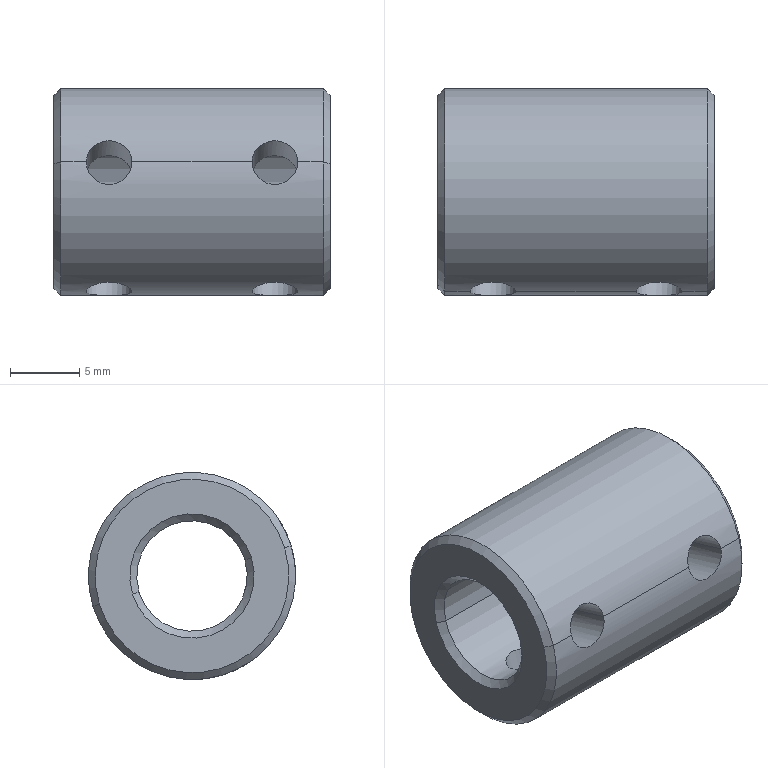Component | SolidWorks | 04-004CouplingSleeve-1 | 1 solid | 22 faces | box 20 x 15 x 15 mm | volume 2390 mm3 | cylinder 12 | cone 8 | plane 2 | commonest cylinder face diameters 3.3 x8 8 x2 15 x2
build123d program:
from build123d import *

# Parameters (mm, degrees)
SKETCH1_R             = 7.5
SKETCH1_R_2           = 4
BOSS_EXTRUDE1_DEPTH   = 20
M4_TAPPED_HOLE1_D     = 3.3
M4_TAPPED_HOLE1_DEPTH = 6
M4_TAPPED_HOLE1_TIP   = 0.9914
M4_TAPPED_HOLE2_D     = 3.3
M4_TAPPED_HOLE2_DEPTH = 10.1
M4_TAPPED_HOLE2_TIP   = 0.9914
CHAMFER1_SIZE         = 0.5


with BuildPart() as part:
    # Sketch1 → Boss-Extrude1 (new body)
    with BuildSketch(Plane.XY):
        Circle(SKETCH1_R)
        Circle(SKETCH1_R_2, mode=Mode.SUBTRACT)
    extrude(amount=BOSS_EXTRUDE1_DEPTH)

    # M4 Tapped Hole1
    with Locations(Plane.ZY.offset(7.5)):
        with Locations((4, 0), (16, 0)):
            Hole(M4_TAPPED_HOLE1_D / 2, depth=M4_TAPPED_HOLE1_DEPTH)
            with Locations((0, 0, -(M4_TAPPED_HOLE1_DEPTH + M4_TAPPED_HOLE1_TIP / 2))):  # 118° drill point
                Cone(0, M4_TAPPED_HOLE1_D / 2, M4_TAPPED_HOLE1_TIP, mode=Mode.SUBTRACT)

    # M4 Tapped Hole2
    with Locations(Plane(origin=(0, 7.5, 0), x_dir=(1, 0, 0), z_dir=(0, 1, 0))):
        with Locations((0, -16), (0, -4)):
            Hole(M4_TAPPED_HOLE2_D / 2, depth=M4_TAPPED_HOLE2_DEPTH)
            with Locations((0, 0, -(M4_TAPPED_HOLE2_DEPTH + M4_TAPPED_HOLE2_TIP / 2))):  # 118° drill point
                Cone(0, M4_TAPPED_HOLE2_D / 2, M4_TAPPED_HOLE2_TIP, mode=Mode.SUBTRACT)

    # Chamfer1
    chamfer1_edges = [part.edges().sort_by_distance(p)[0] for p in [
        (-7.5, 0, 0),
        (-7.5, 0, 20),
        (-4, 0, 0),
        (-4, 0, 20),
    ]]
    chamfer(chamfer1_edges, length=CHAMFER1_SIZE)


solid = part.part

# Placed as in the assembly
solid = solid.moved(Location((159.726, -5.336, 80.465), (149.395, 90, 13.705)))